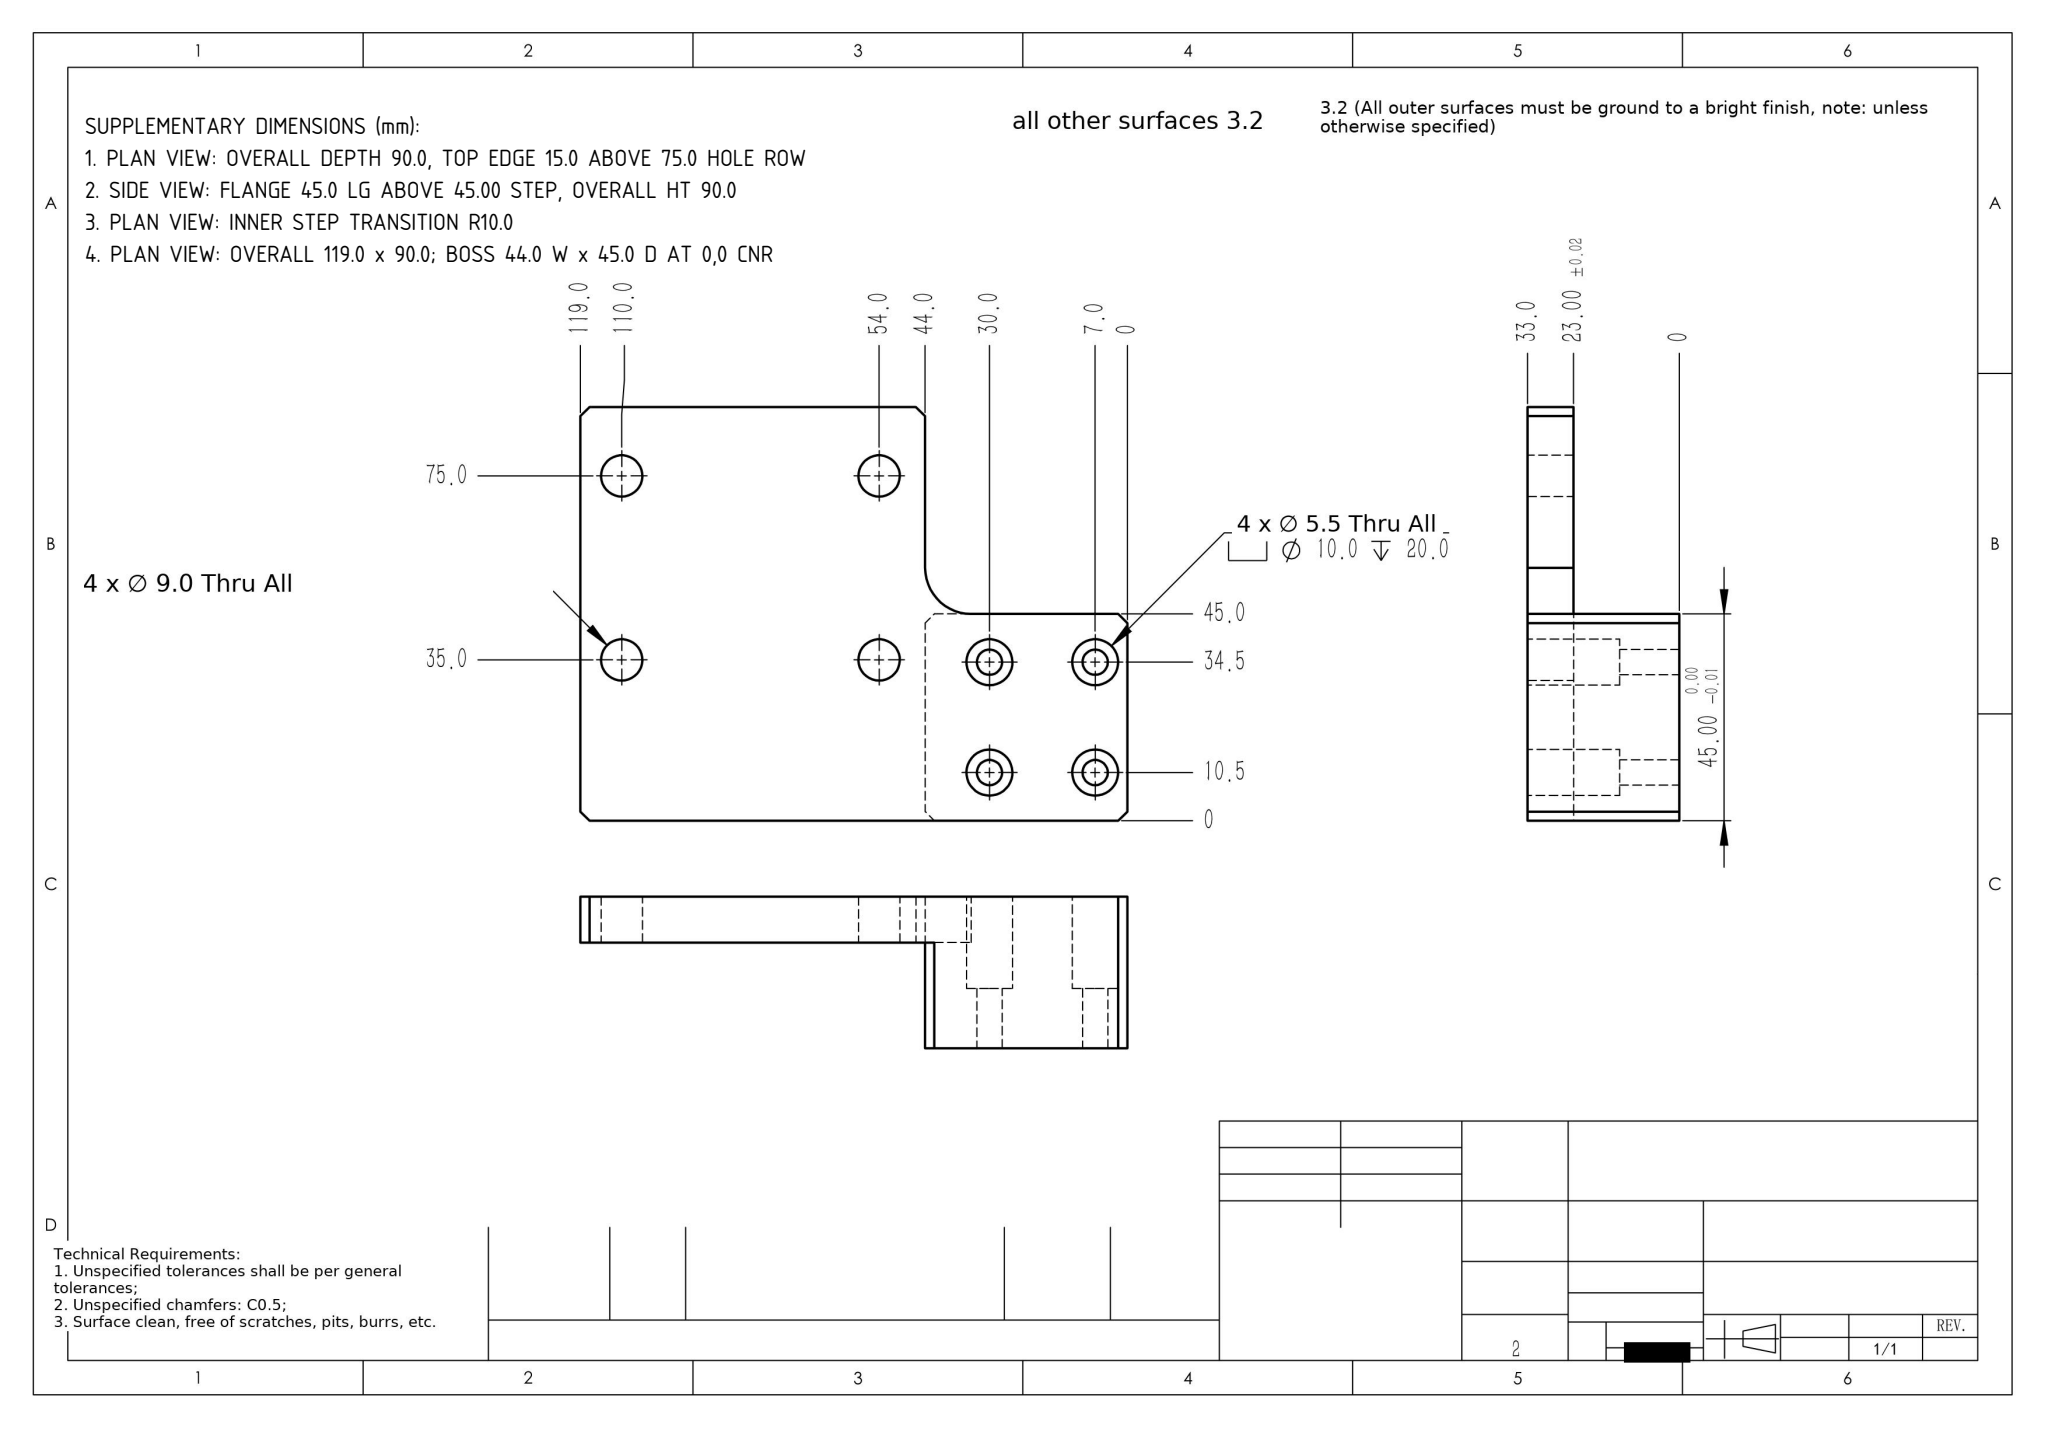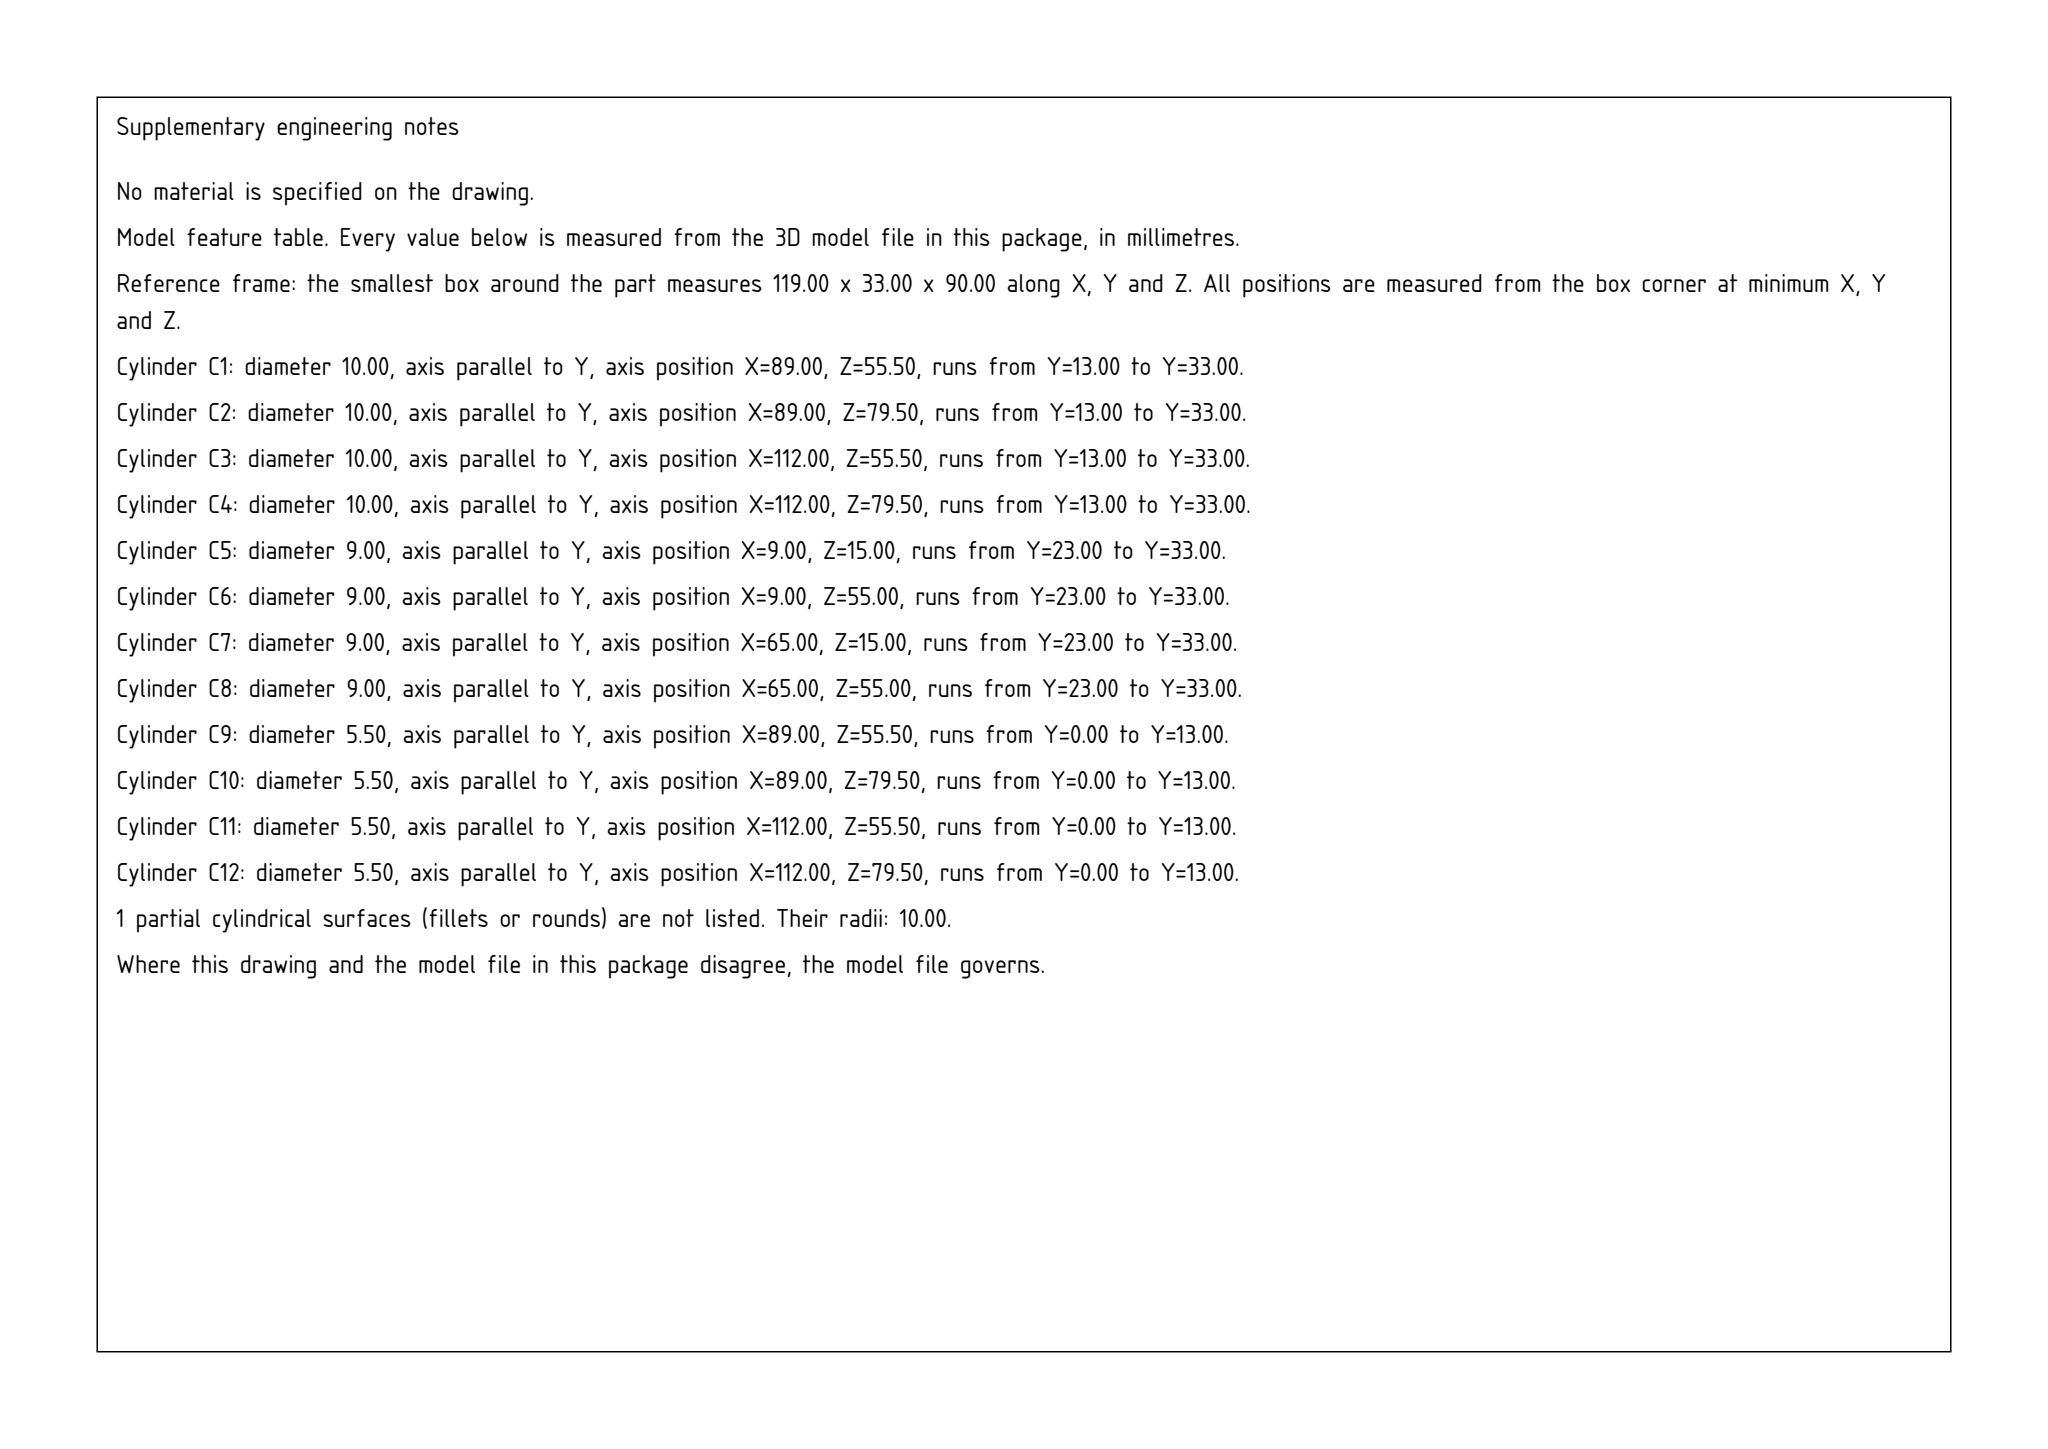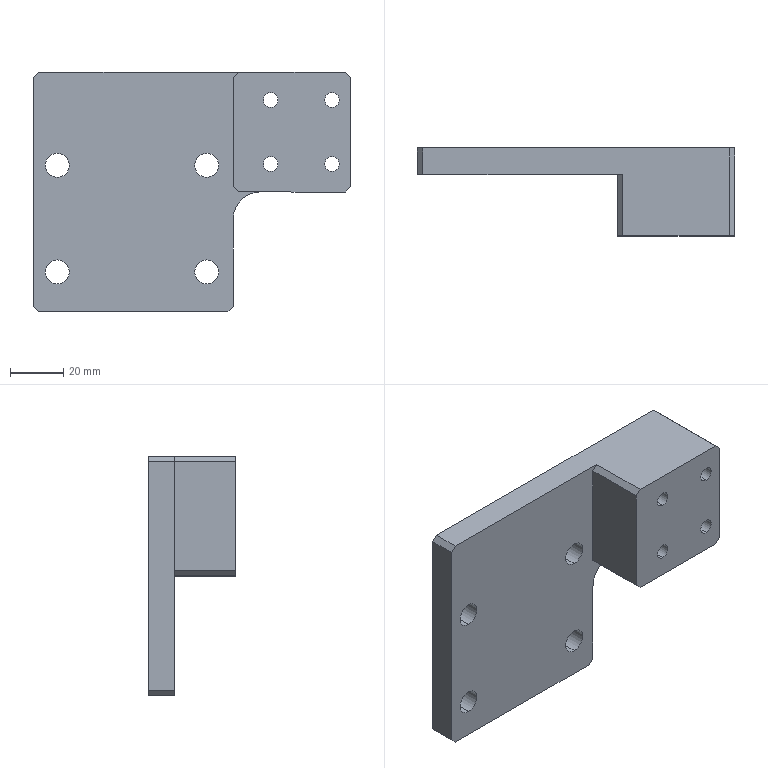Part | SolidWorks | mm | 1 solid | 46 faces | box 119 x 33 x 90 mm | volume 122707 mm3 | cylinder 25 | plane 21 | commonest cylinder face diameters 9 x8 10 x8 5.5 x8 20 x1
build123d program:
from build123d import *

# Parameters (mm, degrees)
SKETCH1_W                                       = 119
SKETCH1_H                                       = 33
BOSS_EXTRUDE1_DEPTH                             = 90
SKETCH2_W                                       = 75
SKETCH2_H                                       = 23
CUT_EXTRUDE1_DEPTH                              = 110.144
M5_HEX_SOCKET_HEAD_CAP_SCREW_CBORE1_D           = 5.5
M5_HEX_SOCKET_HEAD_CAP_SCREW_CBORE1_CBORE_D     = 10
M5_HEX_SOCKET_HEAD_CAP_SCREW_CBORE1_CBORE_DEPTH = 20
M8_CLEARANCE_HOLE1_D                            = 9
SKETCH10_W                                      = 44
SKETCH10_H                                      = 45
CUT_EXTRUDE2_DEPTH                              = 113.824
FILLET1_R                                       = 10
CHAMFER1_SIZE                                   = 2


with BuildPart() as part:
    # Sketch1 → Boss-Extrude1 (new body)
    with BuildSketch(Plane.XY):
        Rectangle(SKETCH1_W, SKETCH1_H)
    extrude(amount=BOSS_EXTRUDE1_DEPTH)

    # Sketch2 → Cut-Extrude1 (cut, through all)
    with BuildSketch(Plane.XY.offset(90)):
        with Locations((-22, -5)):
            Rectangle(SKETCH2_W, SKETCH2_H)
    extrude(amount=-CUT_EXTRUDE1_DEPTH, mode=Mode.SUBTRACT)

    # M5 Hex Socket Head Cap Screw CBORE1 (through all)
    with Locations(Plane(origin=(0, 16.5, 0), x_dir=(1, 0, 0), z_dir=(0, 1, 0))):
        with Locations((29.5, -55.5), (52.5, -55.5), (52.5, -79.5), (29.5, -79.5)):
            CounterBoreHole(M5_HEX_SOCKET_HEAD_CAP_SCREW_CBORE1_D / 2, M5_HEX_SOCKET_HEAD_CAP_SCREW_CBORE1_CBORE_D / 2, M5_HEX_SOCKET_HEAD_CAP_SCREW_CBORE1_CBORE_DEPTH)

    # M8 Clearance Hole1 (through all)
    with Locations(Plane(origin=(0, 16.5, 0), x_dir=(1, 0, 0), z_dir=(0, 1, 0))):
        with Locations((-50.5, -15), (-50.5, -55), (5.5, -55), (5.5, -15)):
            Hole(M8_CLEARANCE_HOLE1_D / 2)

    # Sketch10 → Cut-Extrude2 (cut, through all)
    with BuildSketch(Plane(origin=(0, 16.5, 0), x_dir=(1, 0, 0), z_dir=(0, 1, 0))):
        with Locations((37.5, -22.5)):
            Rectangle(SKETCH10_W, SKETCH10_H)
    extrude(amount=-CUT_EXTRUDE2_DEPTH, mode=Mode.SUBTRACT)

    # Fillet1
    fillet1_edges = [part.edges().sort_by_distance(p)[0] for p in [
        (15.5, 11.5, 45),
    ]]
    fillet(fillet1_edges, radius=FILLET1_R)

    # Chamfer1
    chamfer1_edges = [part.edges().sort_by_distance(p)[0] for p in [
        (-59.5, 11.5, 90),
        (15.5, -5, 90),
        (59.5, 0, 90),
        (-59.5, 11.5, 0),
        (59.5, 0, 45),
        (15.5, -5, 45),
        (15.5, 11.5, 0),
    ]]
    chamfer(chamfer1_edges, length=CHAMFER1_SIZE)


solid = part.part